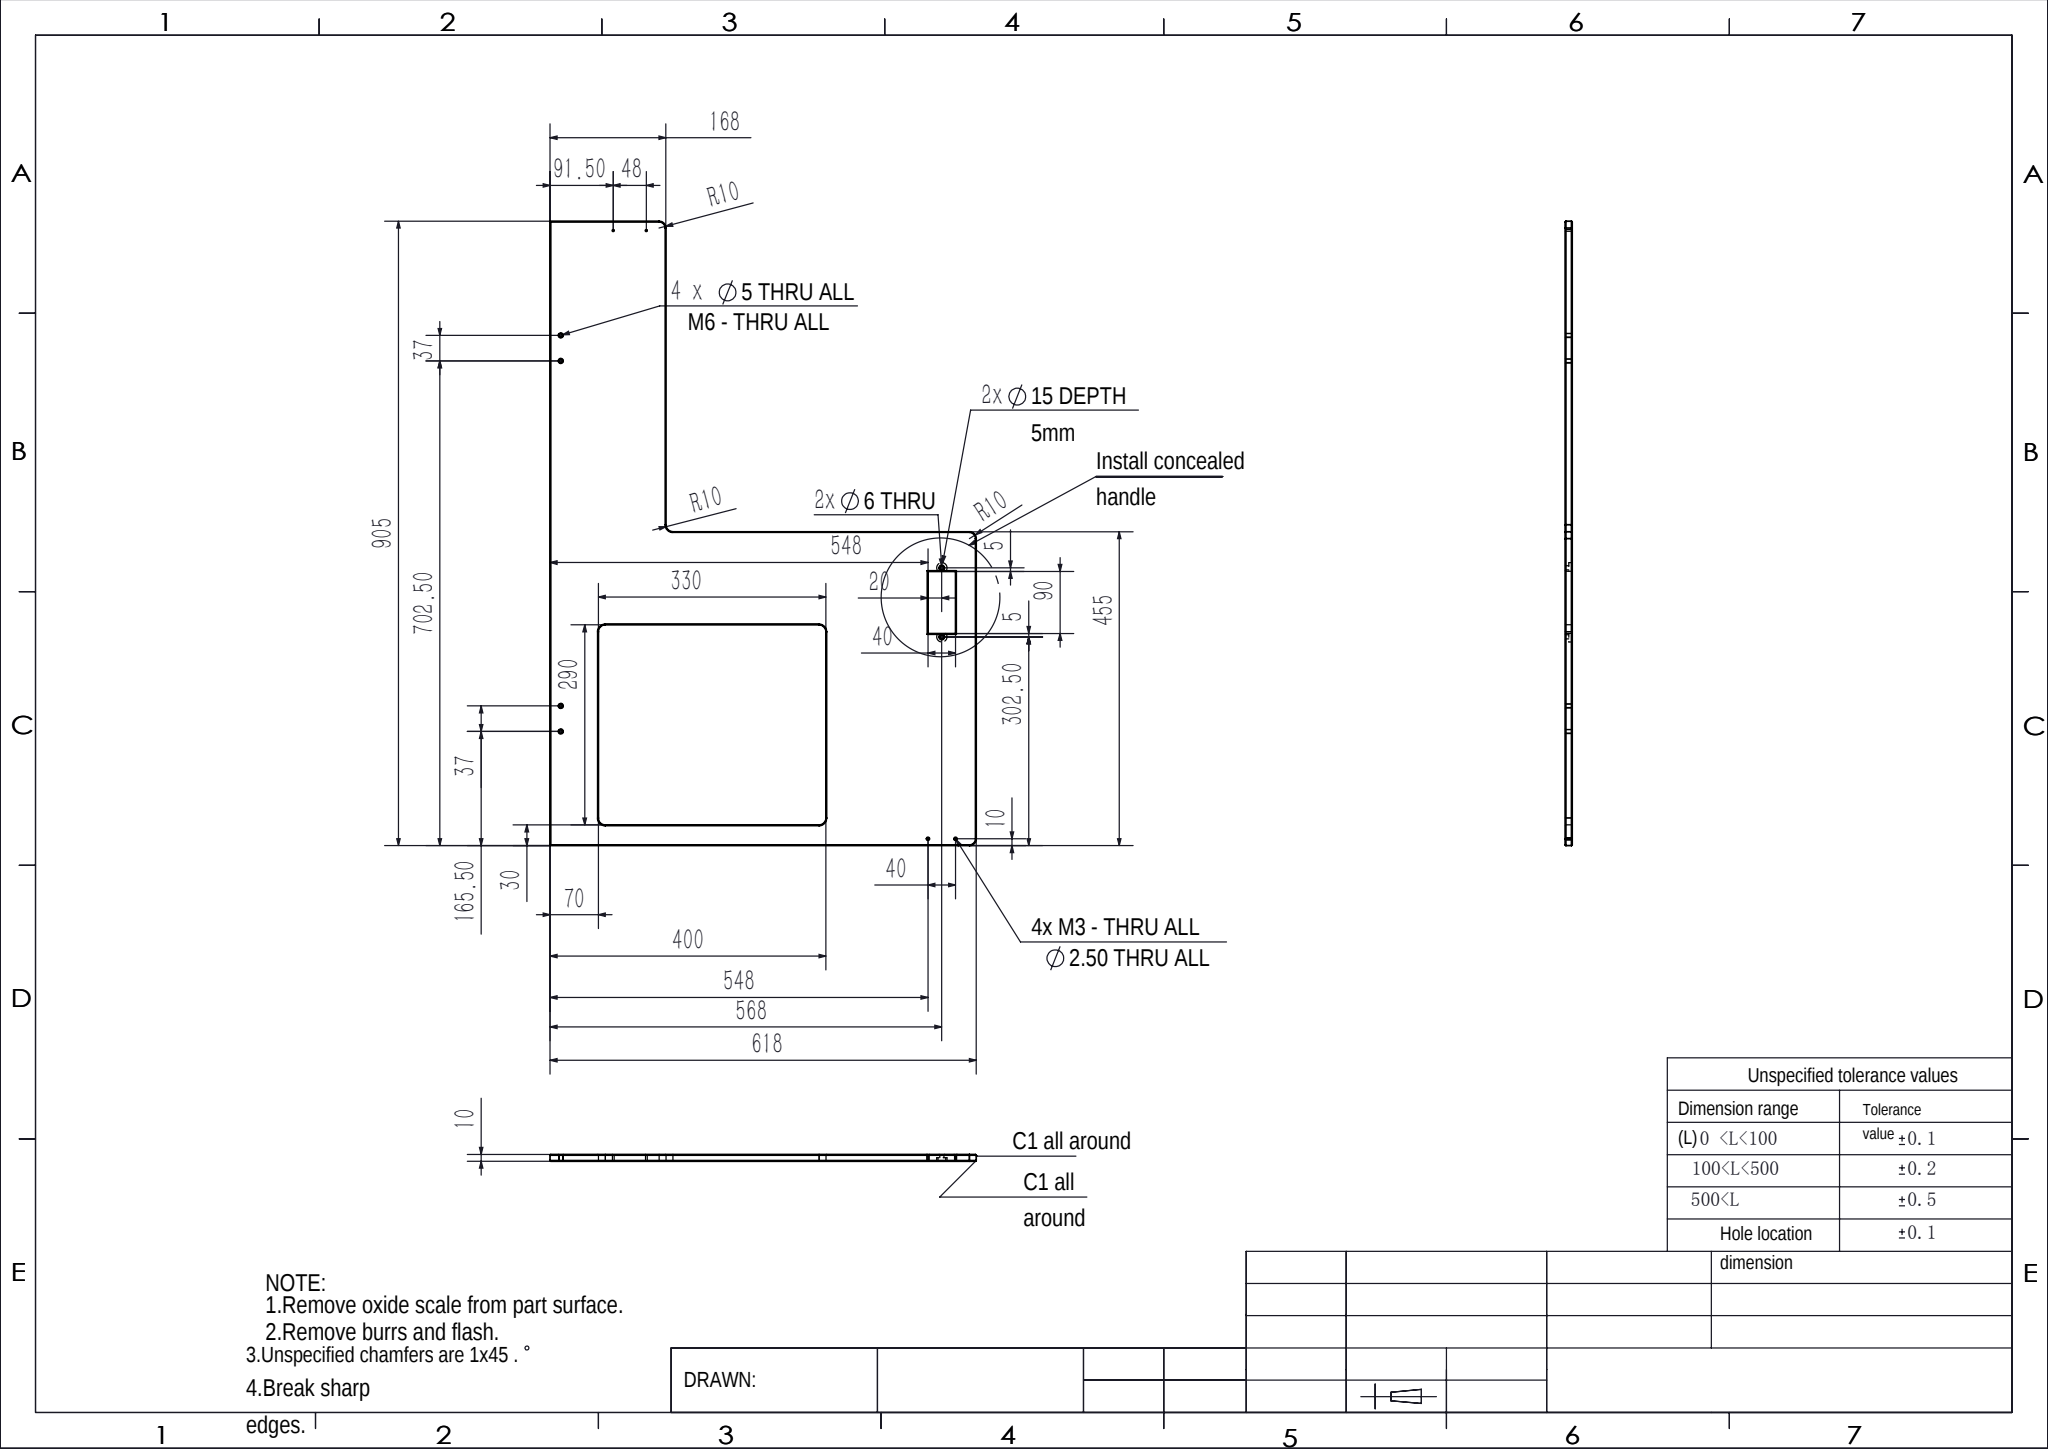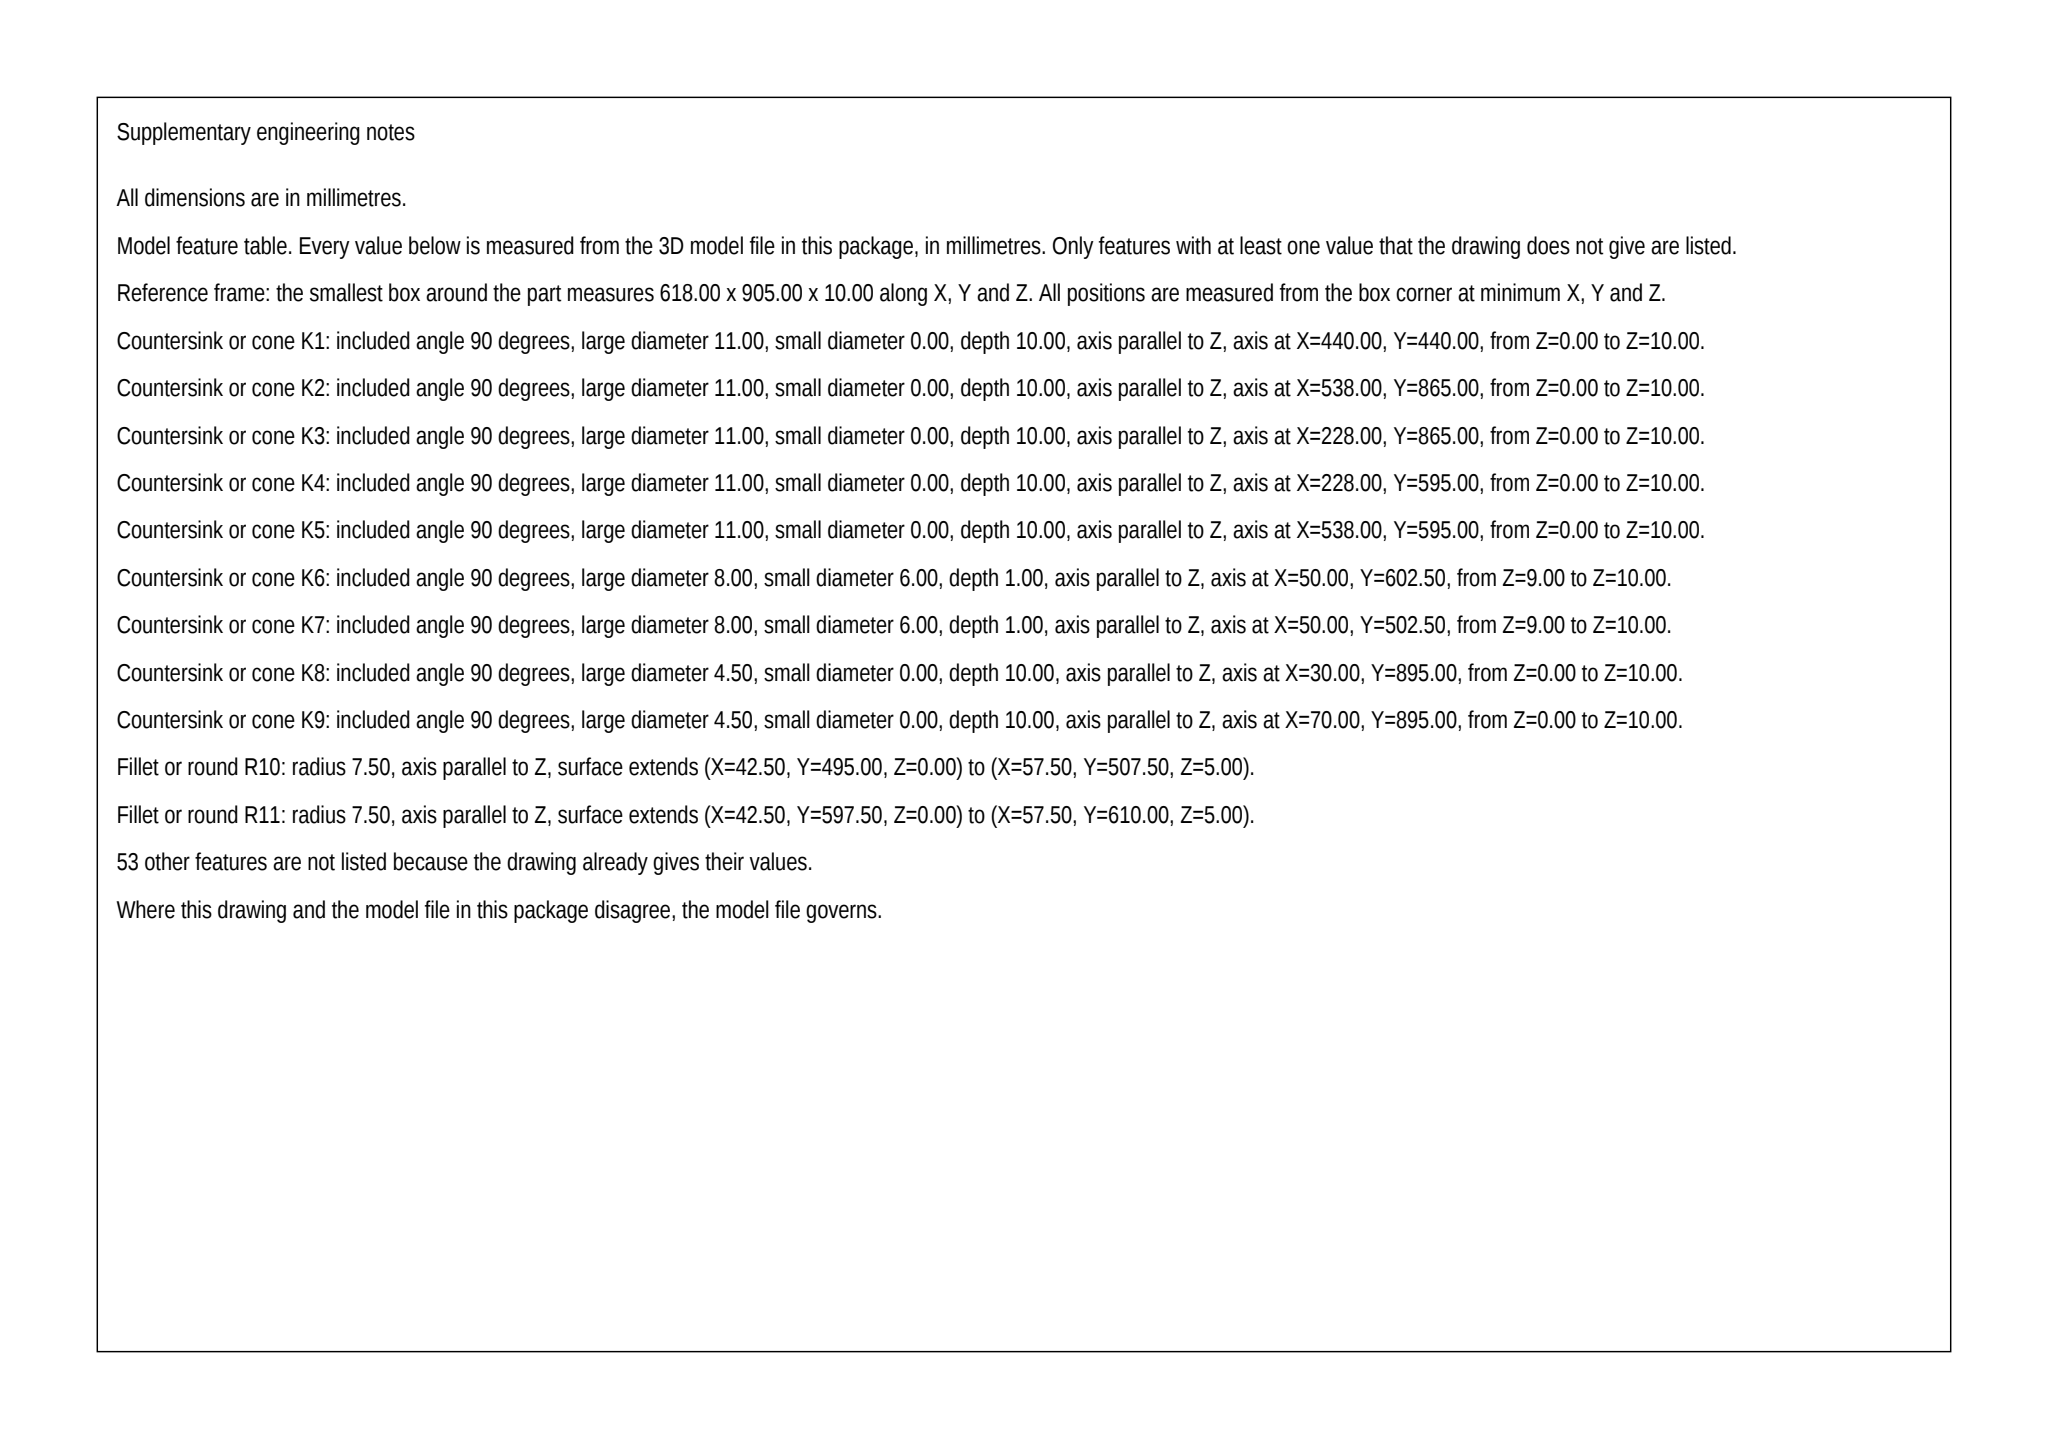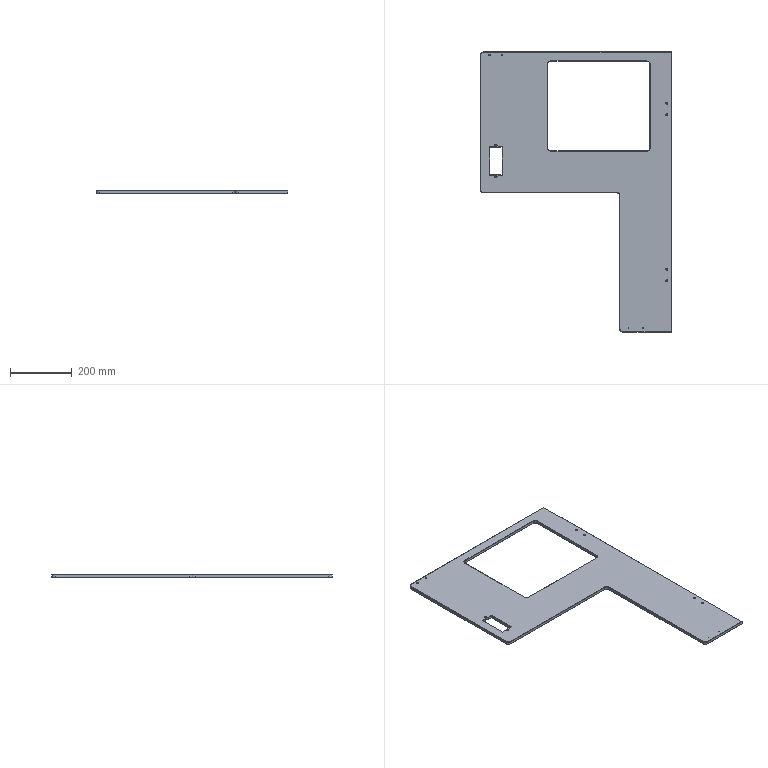Part | SolidWorks | mm | 1 solid | 126 faces | box 618 x 905 x 10 mm | volume 2567877 mm3 | plane 48 | cone 44 | cylinder 34 | commonest cylinder face diameters 2.5 x8 5 x8 20 x8 15 x6 6 x4
Drawing notes:
4X Ø5 M6 THRU: 15.5 FM RH EDGE; Y=165.5, 202.5, 702.5, 739.5 FM BTM | from the solid: Ø5 z-cyls at x=602.5 (618-602.5=15.5), y=165.5/202.5/702.5/739.5; bbox 618x905x10
2X Ø6 THRU, CBORE Ø15 DP 5: 50 FM LH EDGE; 502.5 & 602.5 FM BTM | from the solid: Ø6 thru + Ø15 DP 5 z-cyls at (50,502.5) and (50,602.5)
4X M3 THRU: 30 & 70 FM LH EDGE x 10 FM TOP; 478.5 & 526.5 x 13.5 FM BTM | from the solid: Ø2.5 z-cyls at (30,895),(70,895),(478.5,13.5),(526.5,13.5); bbox 618x905x10
4X R10 AT CORNERS OF 330 X 290 CUTOUT | from the solid: R10 cyls (dia 20, axis z) at (228,595),(228,865),(538,595),(538,865); cutout x218-548 (330), y585-875 (290)
R10 AT LOWER RH CORNER OF PLATE | from the solid: R10 cyl (dia 20, axis z) at model (10,895) = drawing lower-right corner, 10 from both outer edges (x=0/618, y=0/905)
40 X 90 CONCEALED HANDLE SLOT DP 5, NOT THRU | from the solid: Slot planes x=30/70 (40 wide), y=507.5/597.5 (90), bottom plane z=5 in 10 thk plate; 2X O6 THRU remainder